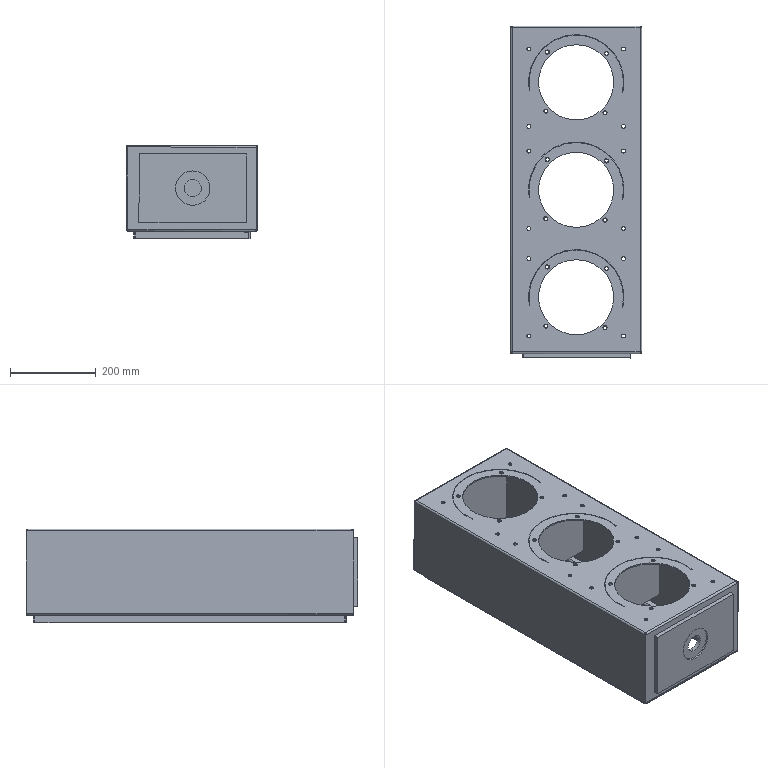Component | SolidWorks | Light-1_LightBox-1 | 1 solid | 247 faces | volume 2470172 mm3 | cylinder 98 | plane 83 | spline 40 | cone 26 | commonest cylinder face diameters 8 x36 9 x24 2 x16 222.1 x6 219.9 x6 175 x6 40 x2 80 x2